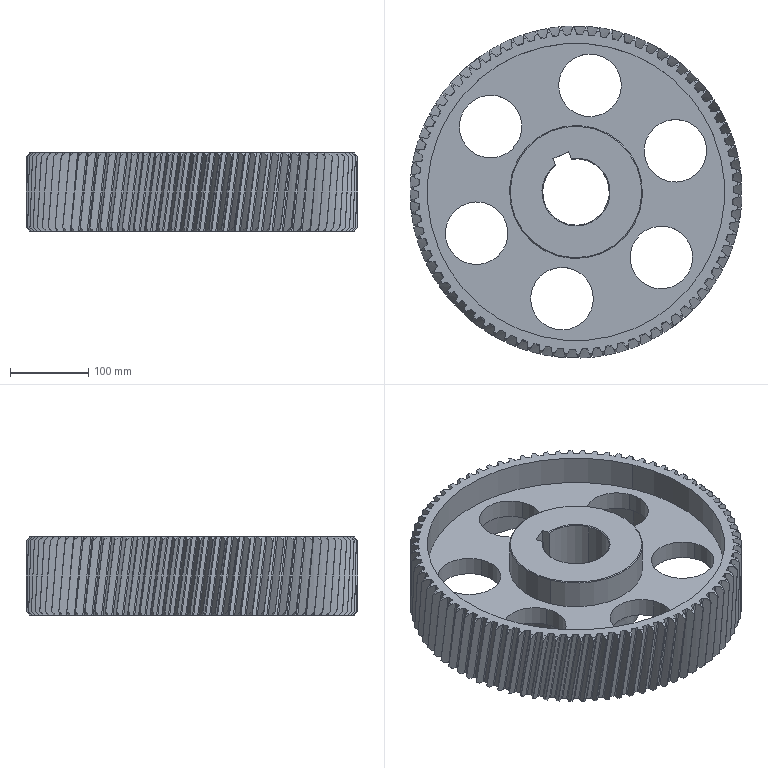Component | SolidWorks | PartAssemblyInLowerHousing-1_LowSpeedAxisAssembly-1_InvoluteLargeGear-1 | 1 solid | 699 faces | volume 4768467 mm3 | spline 410 | cone 178 | cylinder 102 | plane 9 | commonest cylinder face diameters 424.15 x83 80 x12 85 x3 170 x2 380 x2 | material Brass